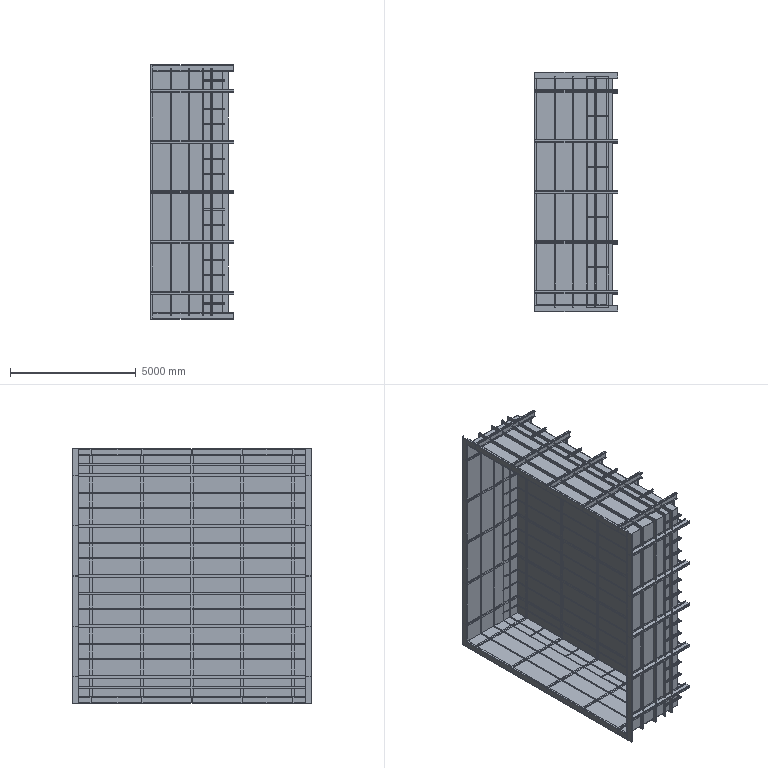Assembly | NX | mm | 89 component files | 117 solids | 3725 faces | box 3300 x 9500 x 10100 mm | volume 2457122580 mm3 | plane 3725
Bill of materials:
unnamed part 1 | 5 |  | Long straight member with an H/I-type cross-section (two parallel flanges joined by a central web), with small notches repeated at regular intervals along its length.
unnamed part 2 | 18 |  | Very long, slender, straight member with a U-shaped channel cross-section and no visible holes or cutouts.
unnamed part 3 | 20 |  | Long straight I-beam-shaped member (tall web between two wide flanges), with four small notches or cutouts along one flange edge at uneven spacing.
unnamed part 4 | 2 |  | Long slender straight member with a C-channel cross-section (web with two short flanges), with small notches repeated at regular intervals along one side.
unnamed part 5 | 5 |  | Long straight member with an H-type cross-section (two parallel flanges joined by a central web). Faint transverse lines appear at regular intervals, but there are no visible cutouts.
unnamed part 6 | 8 |  | Long, very slender, straight member with a C-channel cross-section and no visible holes, notches or other features.
unnamed part 7 | 2 |  | Long straight C-channel-shaped member. Both flanges are interrupted by short gaps at regular intervals, while the web appears to stay continuous.
unnamed part 8 | 1 |  | Solid rectangular block or thick plate with plain flat faces and no visible holes, chamfers or other features.
unnamed part 9 | 28 |  | Straight C-channel-shaped member that appears as two in-line channel segments separated by a small gap. At the segment ends the flanges and web are stepped or offset.
Mates:
1. touch align | chunshuijincao_caogang3 15 face | chunshuijincao_caogang1 1 face
2. touch align | chunshuijincao_caogang3 19 face | chunshuijincao_caogang1 1 face